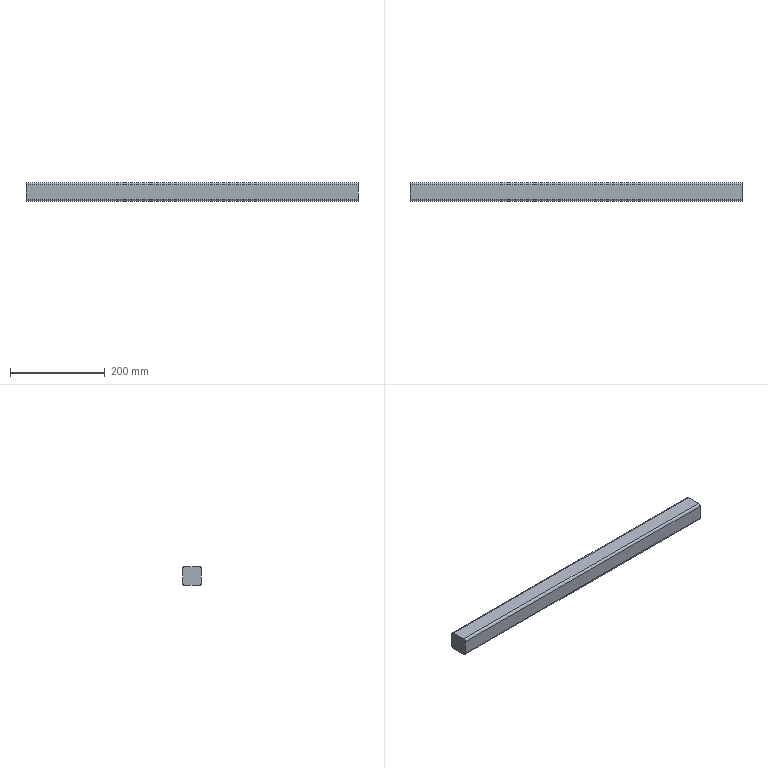Component | SolidWorks | Jig4040-700-2 | 1 solid | 10 faces | box 700 x 40 x 40 mm | volume 1104978 mm3 | plane 6 | cylinder 4 | commonest cylinder face diameters 10 x4 | material Copper
build123d program:
from build123d import *

# Parameters (mm, degrees)
BOSS_EXTRUDE1_DEPTH = 700


with BuildPart() as part:
    # Sketch1 → Boss-Extrude1 (new body)
    with BuildSketch(Plane(origin=(0, 0, 0), x_dir=(0, 0, -1), z_dir=(1, 0, 0))):
        with BuildLine():
            Line((5, 0), (35, 0))
            ThreePointArc((35, 0), (38.536, 1.464), (40, 5))
            Line((40, 5), (40, 35))
            ThreePointArc((40, 35), (38.536, 38.536), (35, 40))
            Line((35, 40), (5, 40))
            ThreePointArc((5, 40), (1.464, 38.536), (0, 35))
            Line((0, 35), (0, 5))
            ThreePointArc((0, 5), (1.464, 1.464), (5, 0))
        make_face()
    extrude(amount=BOSS_EXTRUDE1_DEPTH)


solid = part.part

# Placed as in the assembly
solid = solid.moved(Location((11.992, -17.909, 830), (0, 0, 0)))
STEP:
#1=COLOUR_RGB('',0.7922,0.8196,0.9333);
#2=FILL_AREA_STYLE_COLOUR('',#1);
#3=FILL_AREA_STYLE('',(#2));
#4=SURFACE_STYLE_FILL_AREA(#3);
#5=SURFACE_SIDE_STYLE('',(#4));
#6=SURFACE_STYLE_USAGE(.BOTH.,#5);
#7=PRESENTATION_STYLE_ASSIGNMENT((#6));
#8=CARTESIAN_POINT('',(0.4721,0.8697,32.48));
#9=VERTEX_POINT('',#8);
#10=CARTESIAN_POINT('',(0.4721,0.6729,32.677));
#11=VERTEX_POINT('',#10);
#12=CARTESIAN_POINT('',(0.4721,0.6729,32.48));
#13=DIRECTION('',(1.,0.,0.));
#14=DIRECTION('',(0.,0.,1.));
#15=AXIS2_PLACEMENT_3D('',#12,#13,#14);
#16=CIRCLE('',#15,0.1969);
#17=EDGE_CURVE('',#9,#11,#16,.T.);
#18=ORIENTED_EDGE('',*,*,#17,.T.);
#19=CARTESIAN_POINT('',(28.031,0.6729,32.677));
#20=VERTEX_POINT('',#19);
#21=CARTESIAN_POINT('',(28.031,0.6729,32.677));
#22=DIRECTION('',(-1.,0.,0.));
#23=VECTOR('',#22,39.37);
#24=LINE('',#21,#23);
#25=EDGE_CURVE('',#20,#11,#24,.T.);
#26=ORIENTED_EDGE('',*,*,#25,.F.);
#27=CARTESIAN_POINT('',(28.031,0.8697,32.48));
#28=VERTEX_POINT('',#27);
#29=CARTESIAN_POINT('',(28.031,0.6729,32.48));
#30=DIRECTION('',(1.,0.,0.));
#31=DIRECTION('',(0.,0.,1.));
#32=AXIS2_PLACEMENT_3D('',#29,#30,#31);
#33=CIRCLE('',#32,0.1969);
#34=EDGE_CURVE('',#28,#20,#33,.T.);
#35=ORIENTED_EDGE('',*,*,#34,.F.);
#36=CARTESIAN_POINT('',(28.031,0.8697,32.48));
#37=DIRECTION('',(-1.,0.,0.));
#38=VECTOR('',#37,39.37);
#39=LINE('',#36,#38);
#40=EDGE_CURVE('',#28,#9,#39,.T.);
#41=ORIENTED_EDGE('',*,*,#40,.T.);
#42=EDGE_LOOP('',(#18,#26,#35,#41));
#43=FACE_OUTER_BOUND('',#42,.T.);
#44=CARTESIAN_POINT('',(28.031,0.6729,32.48));
#45=DIRECTION('',(-1.,0.,0.));
#46=DIRECTION('',(0.,0.,1.));
#47=AXIS2_PLACEMENT_3D('',#44,#45,#46);
#48=CYLINDRICAL_SURFACE('',#47,0.1969);
#49=ADVANCED_FACE('',(#43),#48,.T.);
#50=CARTESIAN_POINT('',(0.4721,-0.5082,32.677));
#51=VERTEX_POINT('',#50);
#52=CARTESIAN_POINT('',(0.4721,-0.5082,32.677));
#53=DIRECTION('',(0.,-1.,0.));
#54=VECTOR('',#53,39.37);
#55=LINE('',#52,#54);
#56=EDGE_CURVE('',#11,#51,#55,.T.);
#57=ORIENTED_EDGE('',*,*,#56,.T.);
#58=CARTESIAN_POINT('',(28.031,-0.5082,32.677));
#59=VERTEX_POINT('',#58);
#60=CARTESIAN_POINT('',(28.031,-0.5082,32.677));
#61=DIRECTION('',(-1.,0.,0.));
#62=VECTOR('',#61,39.37);
#63=LINE('',#60,#62);
#64=EDGE_CURVE('',#59,#51,#63,.T.);
#65=ORIENTED_EDGE('',*,*,#64,.F.);
#66=CARTESIAN_POINT('',(28.031,-0.5082,32.677));
#67=DIRECTION('',(0.,-1.,0.));
#68=VECTOR('',#67,39.37);
#69=LINE('',#66,#68);
#70=EDGE_CURVE('',#20,#59,#69,.T.);
#71=ORIENTED_EDGE('',*,*,#70,.F.);
#72=ORIENTED_EDGE('',*,*,#25,.T.);
#73=EDGE_LOOP('',(#57,#65,#71,#72));
#74=FACE_OUTER_BOUND('',#73,.T.);
#75=CARTESIAN_POINT('',(28.031,-0.5082,32.677));
#76=DIRECTION('',(0.,0.,-1.));
#77=DIRECTION('',(-1.,0.,0.));
#78=AXIS2_PLACEMENT_3D('',#75,#76,#77);
#79=PLANE('',#78);
#80=ADVANCED_FACE('',(#74),#79,.F.);
#81=CARTESIAN_POINT('',(0.4721,-0.7051,32.48));
#82=VERTEX_POINT('',#81);
#83=CARTESIAN_POINT('',(0.4721,-0.5082,32.48));
#84=DIRECTION('',(1.,0.,0.));
#85=DIRECTION('',(0.,0.,-1.));
#86=AXIS2_PLACEMENT_3D('',#83,#84,#85);
#87=CIRCLE('',#86,0.1969);
#88=EDGE_CURVE('',#51,#82,#87,.T.);
#89=ORIENTED_EDGE('',*,*,#88,.T.);
#90=CARTESIAN_POINT('',(28.031,-0.7051,32.48));
#91=VERTEX_POINT('',#90);
#92=CARTESIAN_POINT('',(28.031,-0.7051,32.48));
#93=DIRECTION('',(-1.,0.,0.));
#94=VECTOR('',#93,39.37);
#95=LINE('',#92,#94);
#96=EDGE_CURVE('',#91,#82,#95,.T.);
#97=ORIENTED_EDGE('',*,*,#96,.F.);
#98=CARTESIAN_POINT('',(28.031,-0.5082,32.48));
#99=DIRECTION('',(1.,0.,0.));
#100=DIRECTION('',(0.,0.,-1.));
#101=AXIS2_PLACEMENT_3D('',#98,#99,#100);
#102=CIRCLE('',#101,0.1969);
#103=EDGE_CURVE('',#59,#91,#102,.T.);
#104=ORIENTED_EDGE('',*,*,#103,.F.);
#105=ORIENTED_EDGE('',*,*,#64,.T.);
#106=EDGE_LOOP('',(#89,#97,#104,#105));
#107=FACE_OUTER_BOUND('',#106,.T.);
#108=CARTESIAN_POINT('',(28.031,-0.5082,32.48));
#109=DIRECTION('',(-1.,0.,0.));
#110=DIRECTION('',(0.,0.,1.));
#111=AXIS2_PLACEMENT_3D('',#108,#109,#110);
#112=CYLINDRICAL_SURFACE('',#111,0.1969);
#113=ADVANCED_FACE('',(#107),#112,.T.);
#114=CARTESIAN_POINT('',(0.4721,-0.7051,31.299));
#115=VERTEX_POINT('',#114);
#116=CARTESIAN_POINT('',(0.4721,-0.7051,32.48));
#117=DIRECTION('',(0.,0.,-1.));
#118=VECTOR('',#117,39.37);
#119=LINE('',#116,#118);
#120=EDGE_CURVE('',#82,#115,#119,.T.);
#121=ORIENTED_EDGE('',*,*,#120,.T.);
#122=CARTESIAN_POINT('',(28.031,-0.7051,31.299));
#123=VERTEX_POINT('',#122);
#124=CARTESIAN_POINT('',(28.031,-0.7051,31.299));
#125=DIRECTION('',(-1.,0.,0.));
#126=VECTOR('',#125,39.37);
#127=LINE('',#124,#126);
#128=EDGE_CURVE('',#123,#115,#127,.T.);
#129=ORIENTED_EDGE('',*,*,#128,.F.);
#130=CARTESIAN_POINT('',(28.031,-0.7051,32.48));
#131=DIRECTION('',(0.,0.,-1.));
#132=VECTOR('',#131,39.37);
#133=LINE('',#130,#132);
#134=EDGE_CURVE('',#91,#123,#133,.T.);
#135=ORIENTED_EDGE('',*,*,#134,.F.);
#136=ORIENTED_EDGE('',*,*,#96,.T.);
#137=EDGE_LOOP('',(#121,#129,#135,#136));
#138=FACE_OUTER_BOUND('',#137,.T.);
#139=CARTESIAN_POINT('',(28.031,-0.7051,32.48));
#140=DIRECTION('',(0.,1.,0.));
#141=DIRECTION('',(0.,0.,1.));
#142=AXIS2_PLACEMENT_3D('',#139,#140,#141);
#143=PLANE('',#142);
#144=ADVANCED_FACE('',(#138),#143,.F.);
#145=CARTESIAN_POINT('',(0.4721,-0.5082,31.102));
#146=VERTEX_POINT('',#145);
#147=CARTESIAN_POINT('',(0.4721,-0.5082,31.299));
#148=DIRECTION('',(1.,0.,0.));
#149=DIRECTION('',(0.,0.,-1.));
#150=AXIS2_PLACEMENT_3D('',#147,#148,#149);
#151=CIRCLE('',#150,0.1969);
#152=EDGE_CURVE('',#115,#146,#151,.T.);
#153=ORIENTED_EDGE('',*,*,#152,.T.);
#154=CARTESIAN_POINT('',(28.031,-0.5082,31.102));
#155=VERTEX_POINT('',#154);
#156=CARTESIAN_POINT('',(28.031,-0.5082,31.102));
#157=DIRECTION('',(-1.,0.,0.));
#158=VECTOR('',#157,39.37);
#159=LINE('',#156,#158);
#160=EDGE_CURVE('',#155,#146,#159,.T.);
#161=ORIENTED_EDGE('',*,*,#160,.F.);
#162=CARTESIAN_POINT('',(28.031,-0.5082,31.299));
#163=DIRECTION('',(1.,0.,0.));
#164=DIRECTION('',(0.,0.,-1.));
#165=AXIS2_PLACEMENT_3D('',#162,#163,#164);
#166=CIRCLE('',#165,0.1969);
#167=EDGE_CURVE('',#123,#155,#166,.T.);
#168=ORIENTED_EDGE('',*,*,#167,.F.);
#169=ORIENTED_EDGE('',*,*,#128,.T.);
#170=EDGE_LOOP('',(#153,#161,#168,#169));
#171=FACE_OUTER_BOUND('',#170,.T.);
#172=CARTESIAN_POINT('',(28.031,-0.5082,31.299));
#173=DIRECTION('',(-1.,0.,0.));
#174=DIRECTION('',(0.,0.,1.));
#175=AXIS2_PLACEMENT_3D('',#172,#173,#174);
#176=CYLINDRICAL_SURFACE('',#175,0.1969);
#177=ADVANCED_FACE('',(#171),#176,.T.);
#178=CARTESIAN_POINT('',(0.4721,0.6729,31.102));
#179=VERTEX_POINT('',#178);
#180=CARTESIAN_POINT('',(0.4721,-0.5082,31.102));
#181=DIRECTION('',(0.,1.,0.));
#182=VECTOR('',#181,39.37);
#183=LINE('',#180,#182);
#184=EDGE_CURVE('',#146,#179,#183,.T.);
#185=ORIENTED_EDGE('',*,*,#184,.T.);
#186=CARTESIAN_POINT('',(28.031,0.6729,31.102));
#187=VERTEX_POINT('',#186);
#188=CARTESIAN_POINT('',(28.031,0.6729,31.102));
#189=DIRECTION('',(-1.,0.,0.));
#190=VECTOR('',#189,39.37);
#191=LINE('',#188,#190);
#192=EDGE_CURVE('',#187,#179,#191,.T.);
#193=ORIENTED_EDGE('',*,*,#192,.F.);
#194=CARTESIAN_POINT('',(28.031,-0.5082,31.102));
#195=DIRECTION('',(0.,1.,0.));
#196=VECTOR('',#195,39.37);
#197=LINE('',#194,#196);
#198=EDGE_CURVE('',#155,#187,#197,.T.);
#199=ORIENTED_EDGE('',*,*,#198,.F.);
#200=ORIENTED_EDGE('',*,*,#160,.T.);
#201=EDGE_LOOP('',(#185,#193,#199,#200));
#202=FACE_OUTER_BOUND('',#201,.T.);
#203=CARTESIAN_POINT('',(28.031,-0.5082,31.102));
#204=DIRECTION('',(0.,0.,1.));
#205=DIRECTION('',(1.,0.,0.));
#206=AXIS2_PLACEMENT_3D('',#203,#204,#205);
#207=PLANE('',#206);
#208=ADVANCED_FACE('',(#202),#207,.F.);
#209=CARTESIAN_POINT('',(0.4721,0.8697,31.299));
#210=VERTEX_POINT('',#209);
#211=CARTESIAN_POINT('',(0.4721,0.6729,31.299));
#212=DIRECTION('',(1.,0.,0.));
#213=DIRECTION('',(0.,0.,-1.));
#214=AXIS2_PLACEMENT_3D('',#211,#212,#213);
#215=CIRCLE('',#214,0.1969);
#216=EDGE_CURVE('',#179,#210,#215,.T.);
#217=ORIENTED_EDGE('',*,*,#216,.T.);
#218=CARTESIAN_POINT('',(28.031,0.8697,31.299));
#219=VERTEX_POINT('',#218);
#220=CARTESIAN_POINT('',(28.031,0.8697,31.299));
#221=DIRECTION('',(-1.,0.,0.));
#222=VECTOR('',#221,39.37);
#223=LINE('',#220,#222);
#224=EDGE_CURVE('',#219,#210,#223,.T.);
#225=ORIENTED_EDGE('',*,*,#224,.F.);
#226=CARTESIAN_POINT('',(28.031,0.6729,31.299));
#227=DIRECTION('',(1.,0.,0.));
#228=DIRECTION('',(0.,0.,-1.));
#229=AXIS2_PLACEMENT_3D('',#226,#227,#228);
#230=CIRCLE('',#229,0.1969);
#231=EDGE_CURVE('',#187,#219,#230,.T.);
#232=ORIENTED_EDGE('',*,*,#231,.F.);
#233=ORIENTED_EDGE('',*,*,#192,.T.);
#234=EDGE_LOOP('',(#217,#225,#232,#233));
#235=FACE_OUTER_BOUND('',#234,.T.);
#236=CARTESIAN_POINT('',(28.031,0.6729,31.299));
#237=DIRECTION('',(-1.,0.,0.));
#238=DIRECTION('',(0.,0.,1.));
#239=AXIS2_PLACEMENT_3D('',#236,#237,#238);
#240=CYLINDRICAL_SURFACE('',#239,0.1969);
#241=ADVANCED_FACE('',(#235),#240,.T.);
#242=CARTESIAN_POINT('',(0.4721,0.8697,32.48));
#243=DIRECTION('',(0.,0.,1.));
#244=VECTOR('',#243,39.37);
#245=LINE('',#242,#244);
#246=EDGE_CURVE('',#210,#9,#245,.T.);
#247=ORIENTED_EDGE('',*,*,#246,.T.);
#248=ORIENTED_EDGE('',*,*,#40,.F.);
#249=CARTESIAN_POINT('',(28.031,0.8697,32.48));
#250=DIRECTION('',(0.,0.,1.));
#251=VECTOR('',#250,39.37);
#252=LINE('',#249,#251);
#253=EDGE_CURVE('',#219,#28,#252,.T.);
#254=ORIENTED_EDGE('',*,*,#253,.F.);
#255=ORIENTED_EDGE('',*,*,#224,.T.);
#256=EDGE_LOOP('',(#247,#248,#254,#255));
#257=FACE_OUTER_BOUND('',#256,.T.);
#258=CARTESIAN_POINT('',(28.031,0.8697,32.48));
#259=DIRECTION('',(0.,-1.,0.));
#260=DIRECTION('',(0.,0.,-1.));
#261=AXIS2_PLACEMENT_3D('',#258,#259,#260);
#262=PLANE('',#261);
#263=ADVANCED_FACE('',(#257),#262,.F.);
#264=ORIENTED_EDGE('',*,*,#34,.T.);
#265=ORIENTED_EDGE('',*,*,#70,.T.);
#266=ORIENTED_EDGE('',*,*,#103,.T.);
#267=ORIENTED_EDGE('',*,*,#134,.T.);
#268=ORIENTED_EDGE('',*,*,#167,.T.);
#269=ORIENTED_EDGE('',*,*,#198,.T.);
#270=ORIENTED_EDGE('',*,*,#231,.T.);
#271=ORIENTED_EDGE('',*,*,#253,.T.);
#272=EDGE_LOOP('',(#264,#265,#266,#267,#268,#269,#270,#271));
#273=FACE_OUTER_BOUND('',#272,.T.);
#274=CARTESIAN_POINT('',(28.031,0.6729,32.48));
#275=DIRECTION('',(-1.,0.,0.));
#276=DIRECTION('',(0.,0.,1.));
#277=AXIS2_PLACEMENT_3D('',#274,#275,#276);
#278=PLANE('',#277);
#279=ADVANCED_FACE('',(#273),#278,.F.);
#280=ORIENTED_EDGE('',*,*,#17,.F.);
#281=ORIENTED_EDGE('',*,*,#246,.F.);
#282=ORIENTED_EDGE('',*,*,#216,.F.);
#283=ORIENTED_EDGE('',*,*,#184,.F.);
#284=ORIENTED_EDGE('',*,*,#152,.F.);
#285=ORIENTED_EDGE('',*,*,#120,.F.);
#286=ORIENTED_EDGE('',*,*,#88,.F.);
#287=ORIENTED_EDGE('',*,*,#56,.F.);
#288=EDGE_LOOP('',(#280,#281,#282,#283,#284,#285,#286,#287));
#289=FACE_OUTER_BOUND('',#288,.T.);
#290=CARTESIAN_POINT('',(0.4721,0.6729,32.48));
#291=DIRECTION('',(-1.,0.,0.));
#292=DIRECTION('',(0.,0.,1.));
#293=AXIS2_PLACEMENT_3D('',#290,#291,#292);
#294=PLANE('',#293);
#295=ADVANCED_FACE('',(#289),#294,.T.);
#296=CLOSED_SHELL('',(#49,#80,#113,#144,#177,#208,#241,#263,#279,#295));
#297=MANIFOLD_SOLID_BREP('',#296);
#298=STYLED_ITEM('',(#7),#297);
#299=(LENGTH_UNIT()NAMED_UNIT(*)SI_UNIT($,.METRE.));
#300=LENGTH_MEASURE_WITH_UNIT(LENGTH_MEASURE(0.0254),#299);
#301=DIMENSIONAL_EXPONENTS(1.,0.,0.,0.,0.,0.,0.);
#302=(CONVERSION_BASED_UNIT('',#300)LENGTH_UNIT()NAMED_UNIT(#301));
#303=UNCERTAINTY_MEASURE_WITH_UNIT(LENGTH_MEASURE(0.00001),#302,'','');
#304=(NAMED_UNIT(*)PLANE_ANGLE_UNIT()SI_UNIT($,.RADIAN.));
#305=(NAMED_UNIT(*)SI_UNIT($,.STERADIAN.)SOLID_ANGLE_UNIT());
#306=(GEOMETRIC_REPRESENTATION_CONTEXT(3)GLOBAL_UNCERTAINTY_ASSIGNED_CONTEXT((#303))GLOBAL_UNIT_ASSIGNED_CONTEXT((#302,#304,#305))REPRESENTATION_CONTEXT('',''));
#307=MECHANICAL_DESIGN_GEOMETRIC_PRESENTATION_REPRESENTATION('',(#298),#306);
#308=CARTESIAN_POINT('',(0.,0.,0.));
#309=DIRECTION('',(0.,0.,1.));
#310=DIRECTION('',(1.,0.,0.));
#311=AXIS2_PLACEMENT_3D('',#308,#309,#310);
#312=(LENGTH_UNIT()NAMED_UNIT(*)SI_UNIT($,.METRE.));
#313=LENGTH_MEASURE_WITH_UNIT(LENGTH_MEASURE(0.0254),#312);
#314=DIMENSIONAL_EXPONENTS(1.,0.,0.,0.,0.,0.,0.);
#315=(CONVERSION_BASED_UNIT('',#313)LENGTH_UNIT()NAMED_UNIT(#314));
#316=UNCERTAINTY_MEASURE_WITH_UNIT(LENGTH_MEASURE(0.00001),#315,'','');
#317=(NAMED_UNIT(*)PLANE_ANGLE_UNIT()SI_UNIT($,.RADIAN.));
#318=(NAMED_UNIT(*)SI_UNIT($,.STERADIAN.)SOLID_ANGLE_UNIT());
#319=(GEOMETRIC_REPRESENTATION_CONTEXT(3)GLOBAL_UNCERTAINTY_ASSIGNED_CONTEXT((#316))GLOBAL_UNIT_ASSIGNED_CONTEXT((#315,#317,#318))REPRESENTATION_CONTEXT('',''));
#320=ADVANCED_BREP_SHAPE_REPRESENTATION('',(#297,#311),#319);
#321=PRESENTATION_LAYER_ASSIGNMENT('','',(#298));